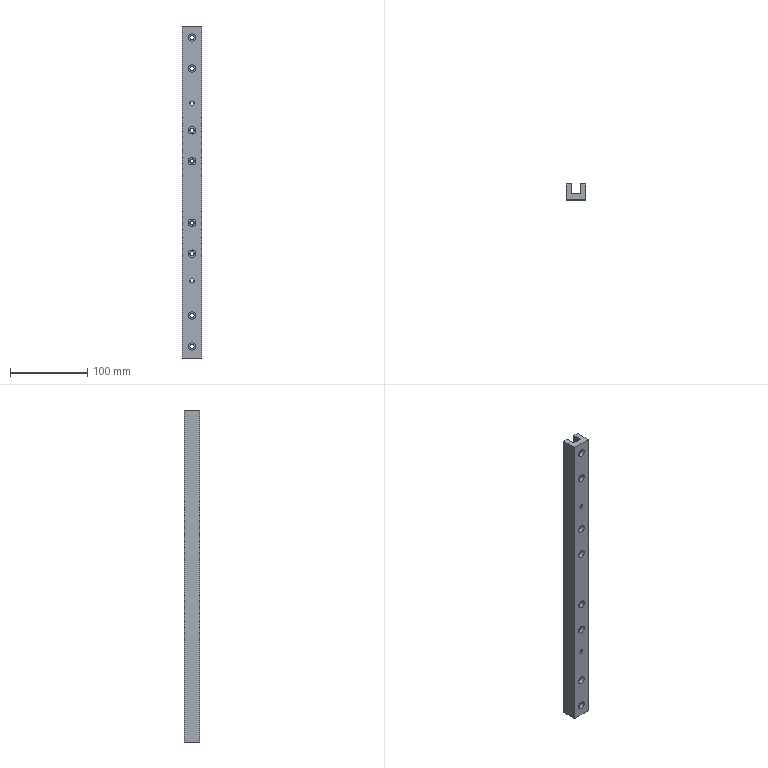Component | SolidWorks | 54-1 | 1 solid | 60 faces | box 25 x 20 x 430 mm | volume 148221 mm3 | cylinder 40 | plane 20 | commonest cylinder face diameters 10 x20 5.5 x20
build123d program:
from build123d import *

# Parameters (mm, degrees)
BOSS_EXTRUDE1_DEPTH                                  = 430
M5_HEX_SOCKET_HEAD_CAP_SCREW_COUNTERBORE_D           = 5.5
M5_HEX_SOCKET_HEAD_CAP_SCREW_COUNTERBORE_CBORE_D     = 10
M5_HEX_SOCKET_HEAD_CAP_SCREW_COUNTERBORE_CBORE_DEPTH = 5.4
M5_HEX_SOCKET_HEAD_CAP_SCREW_COUNTER_2_D             = 5.5
M5_HEX_SOCKET_HEAD_CAP_SCREW_COUNTER_2_CBORE_D       = 10
M5_HEX_SOCKET_HEAD_CAP_SCREW_COUNTER_2_CBORE_DEPTH   = 5.4
LINEAR_PATTERN1_COUNT                                = 4
LINEAR_PATTERN1_PITCH                                = 120


with BuildPart() as part:
    # Sketch1 → Boss-Extrude1 (new body)
    with BuildSketch(Plane.XY):
        Polygon((-6, 8), (6, 8), (6, 20), (12.5, 20), (12.5, 0), (-12.5, 0), (-12.5, 20), (-6, 20), align=None)
    extrude(amount=BOSS_EXTRUDE1_DEPTH)

    # M5 Hex Socket Head Cap Screw Counterbore (through all)
    with Locations(Plane(origin=(0, 8, 0), x_dir=(1, 0, 0), z_dir=(0, 1, 0))):
        with Locations((0, -100), (0, -330)):
            CounterBoreHole(M5_HEX_SOCKET_HEAD_CAP_SCREW_COUNTERBORE_D / 2, M5_HEX_SOCKET_HEAD_CAP_SCREW_COUNTERBORE_CBORE_D / 2, M5_HEX_SOCKET_HEAD_CAP_SCREW_COUNTERBORE_CBORE_DEPTH)

    # M5 Hex Socket Head Cap Screw Counter 2 (through all)
    with Locations(Plane(origin=(0, 0, 0), x_dir=(-1, 0, 0), z_dir=(0, -1, 0))):
        with Locations((0, -15), (0, -55)):
            m5_hex_socket_head_cap_screw_counter_2 = CounterBoreHole(M5_HEX_SOCKET_HEAD_CAP_SCREW_COUNTER_2_D / 2, M5_HEX_SOCKET_HEAD_CAP_SCREW_COUNTER_2_CBORE_D / 2, M5_HEX_SOCKET_HEAD_CAP_SCREW_COUNTER_2_CBORE_DEPTH)

    # Linear Pattern1: M5 Hex Socket Head Cap Screw Counter 2 ×4
    with Locations(*[(0, 0, i * LINEAR_PATTERN1_PITCH) for i in range(1, LINEAR_PATTERN1_COUNT)]):
        add(m5_hex_socket_head_cap_screw_counter_2, mode=Mode.SUBTRACT)


solid = part.part